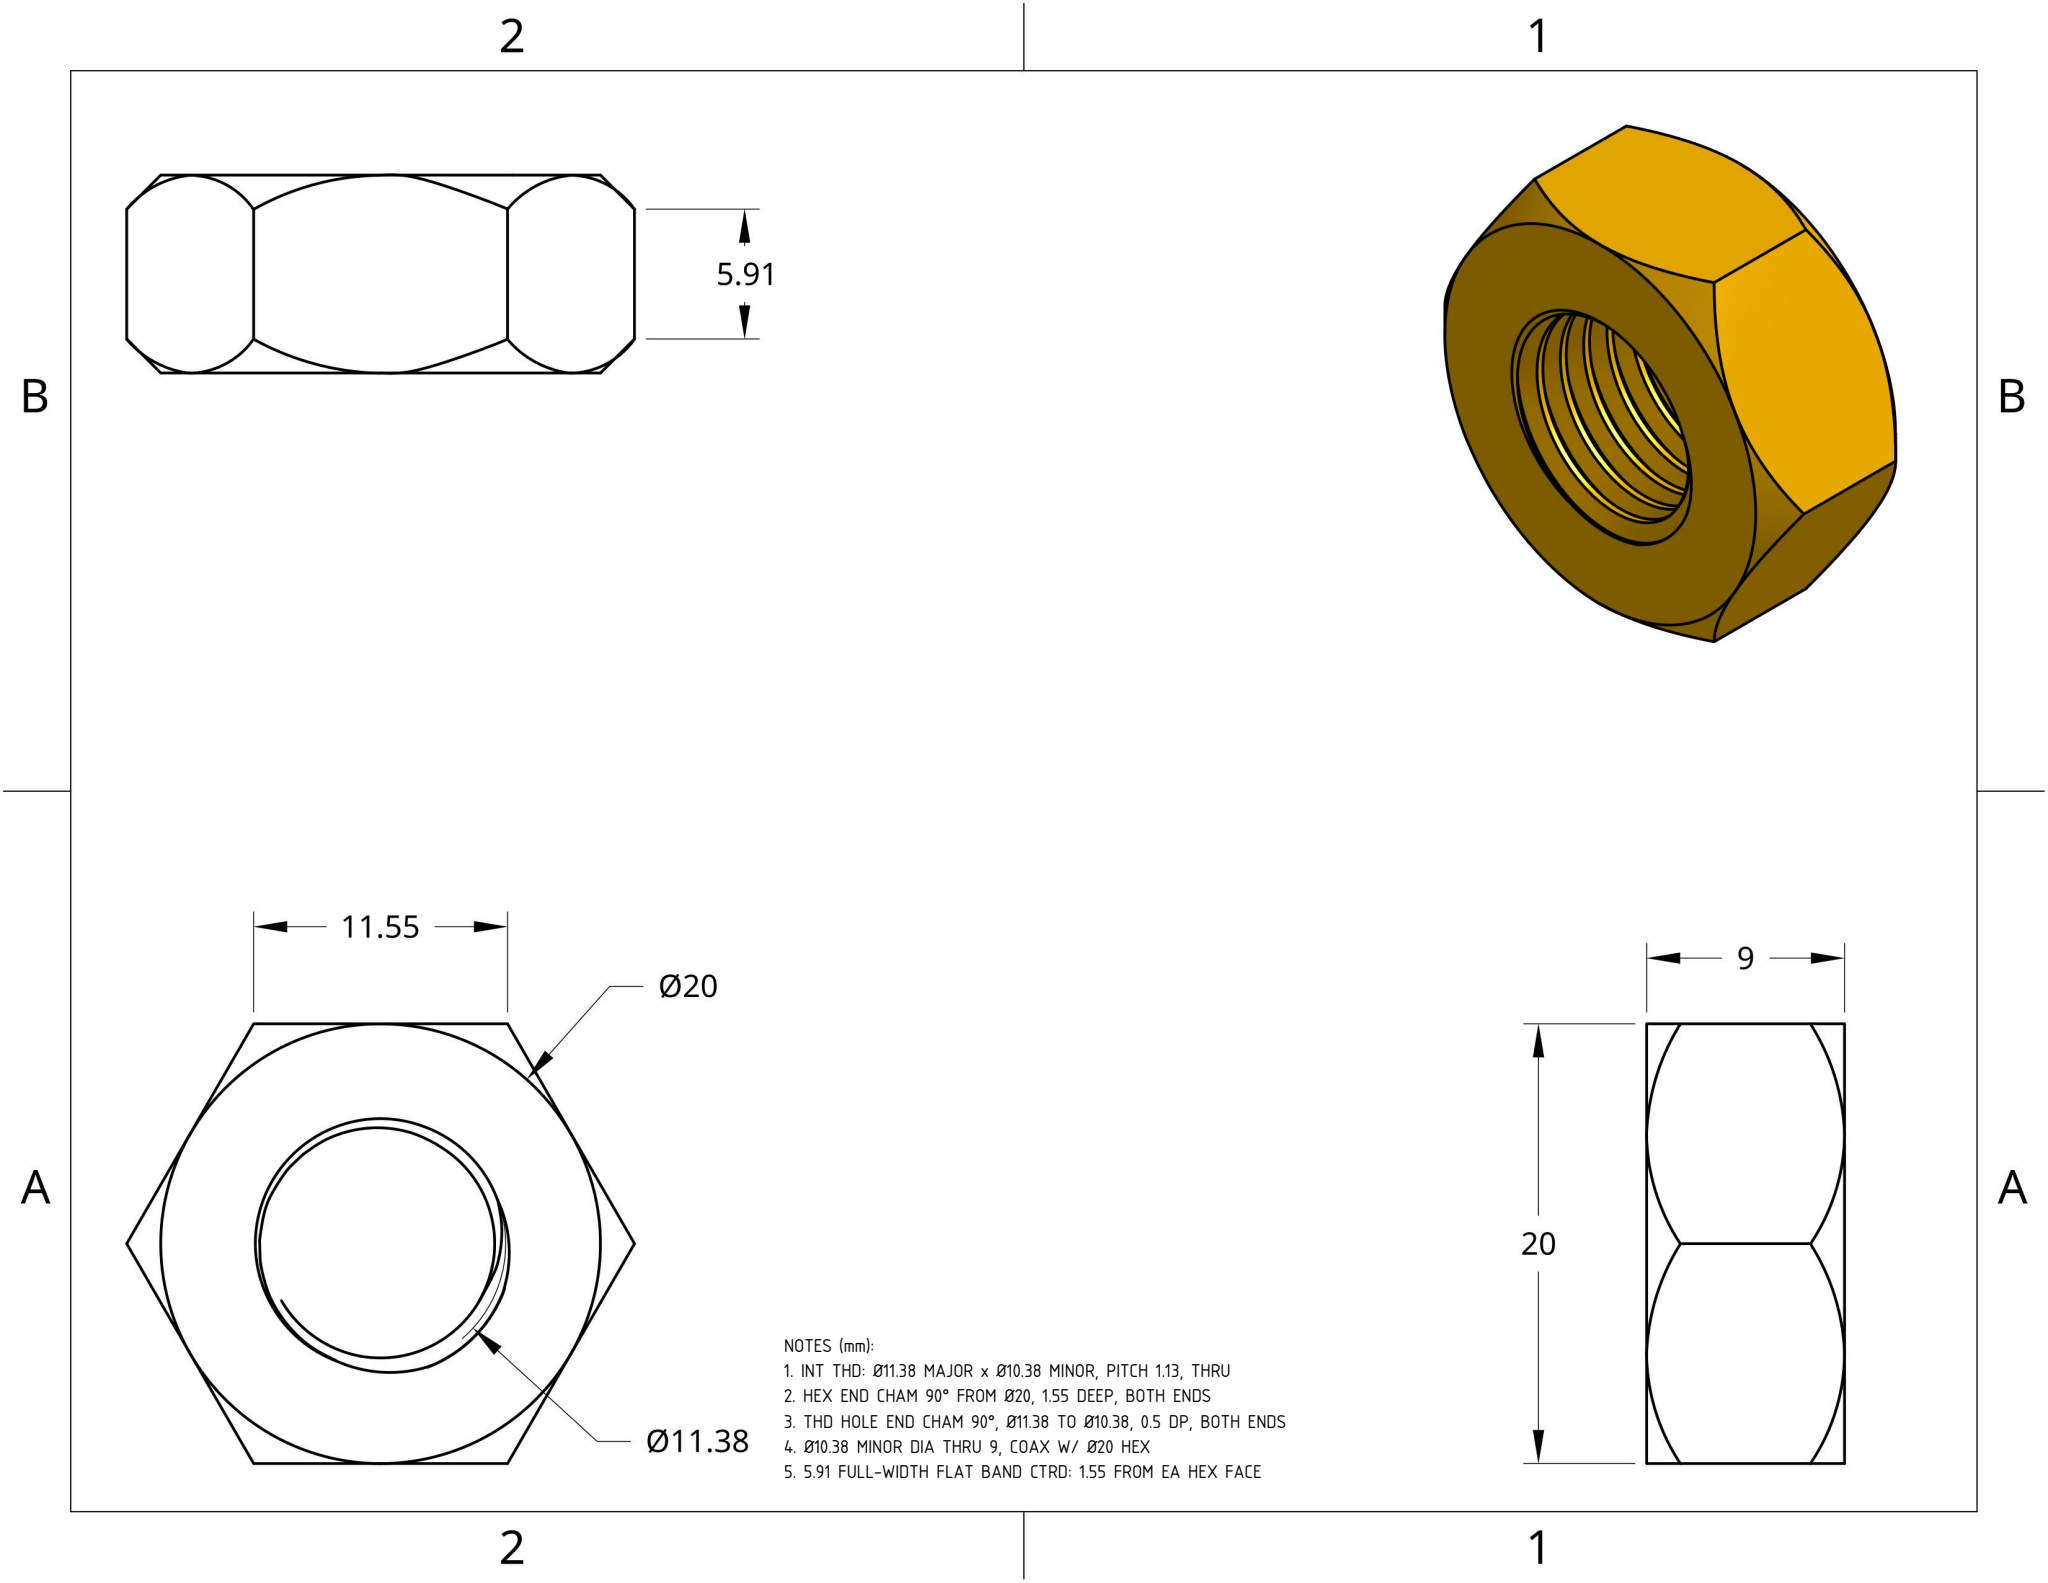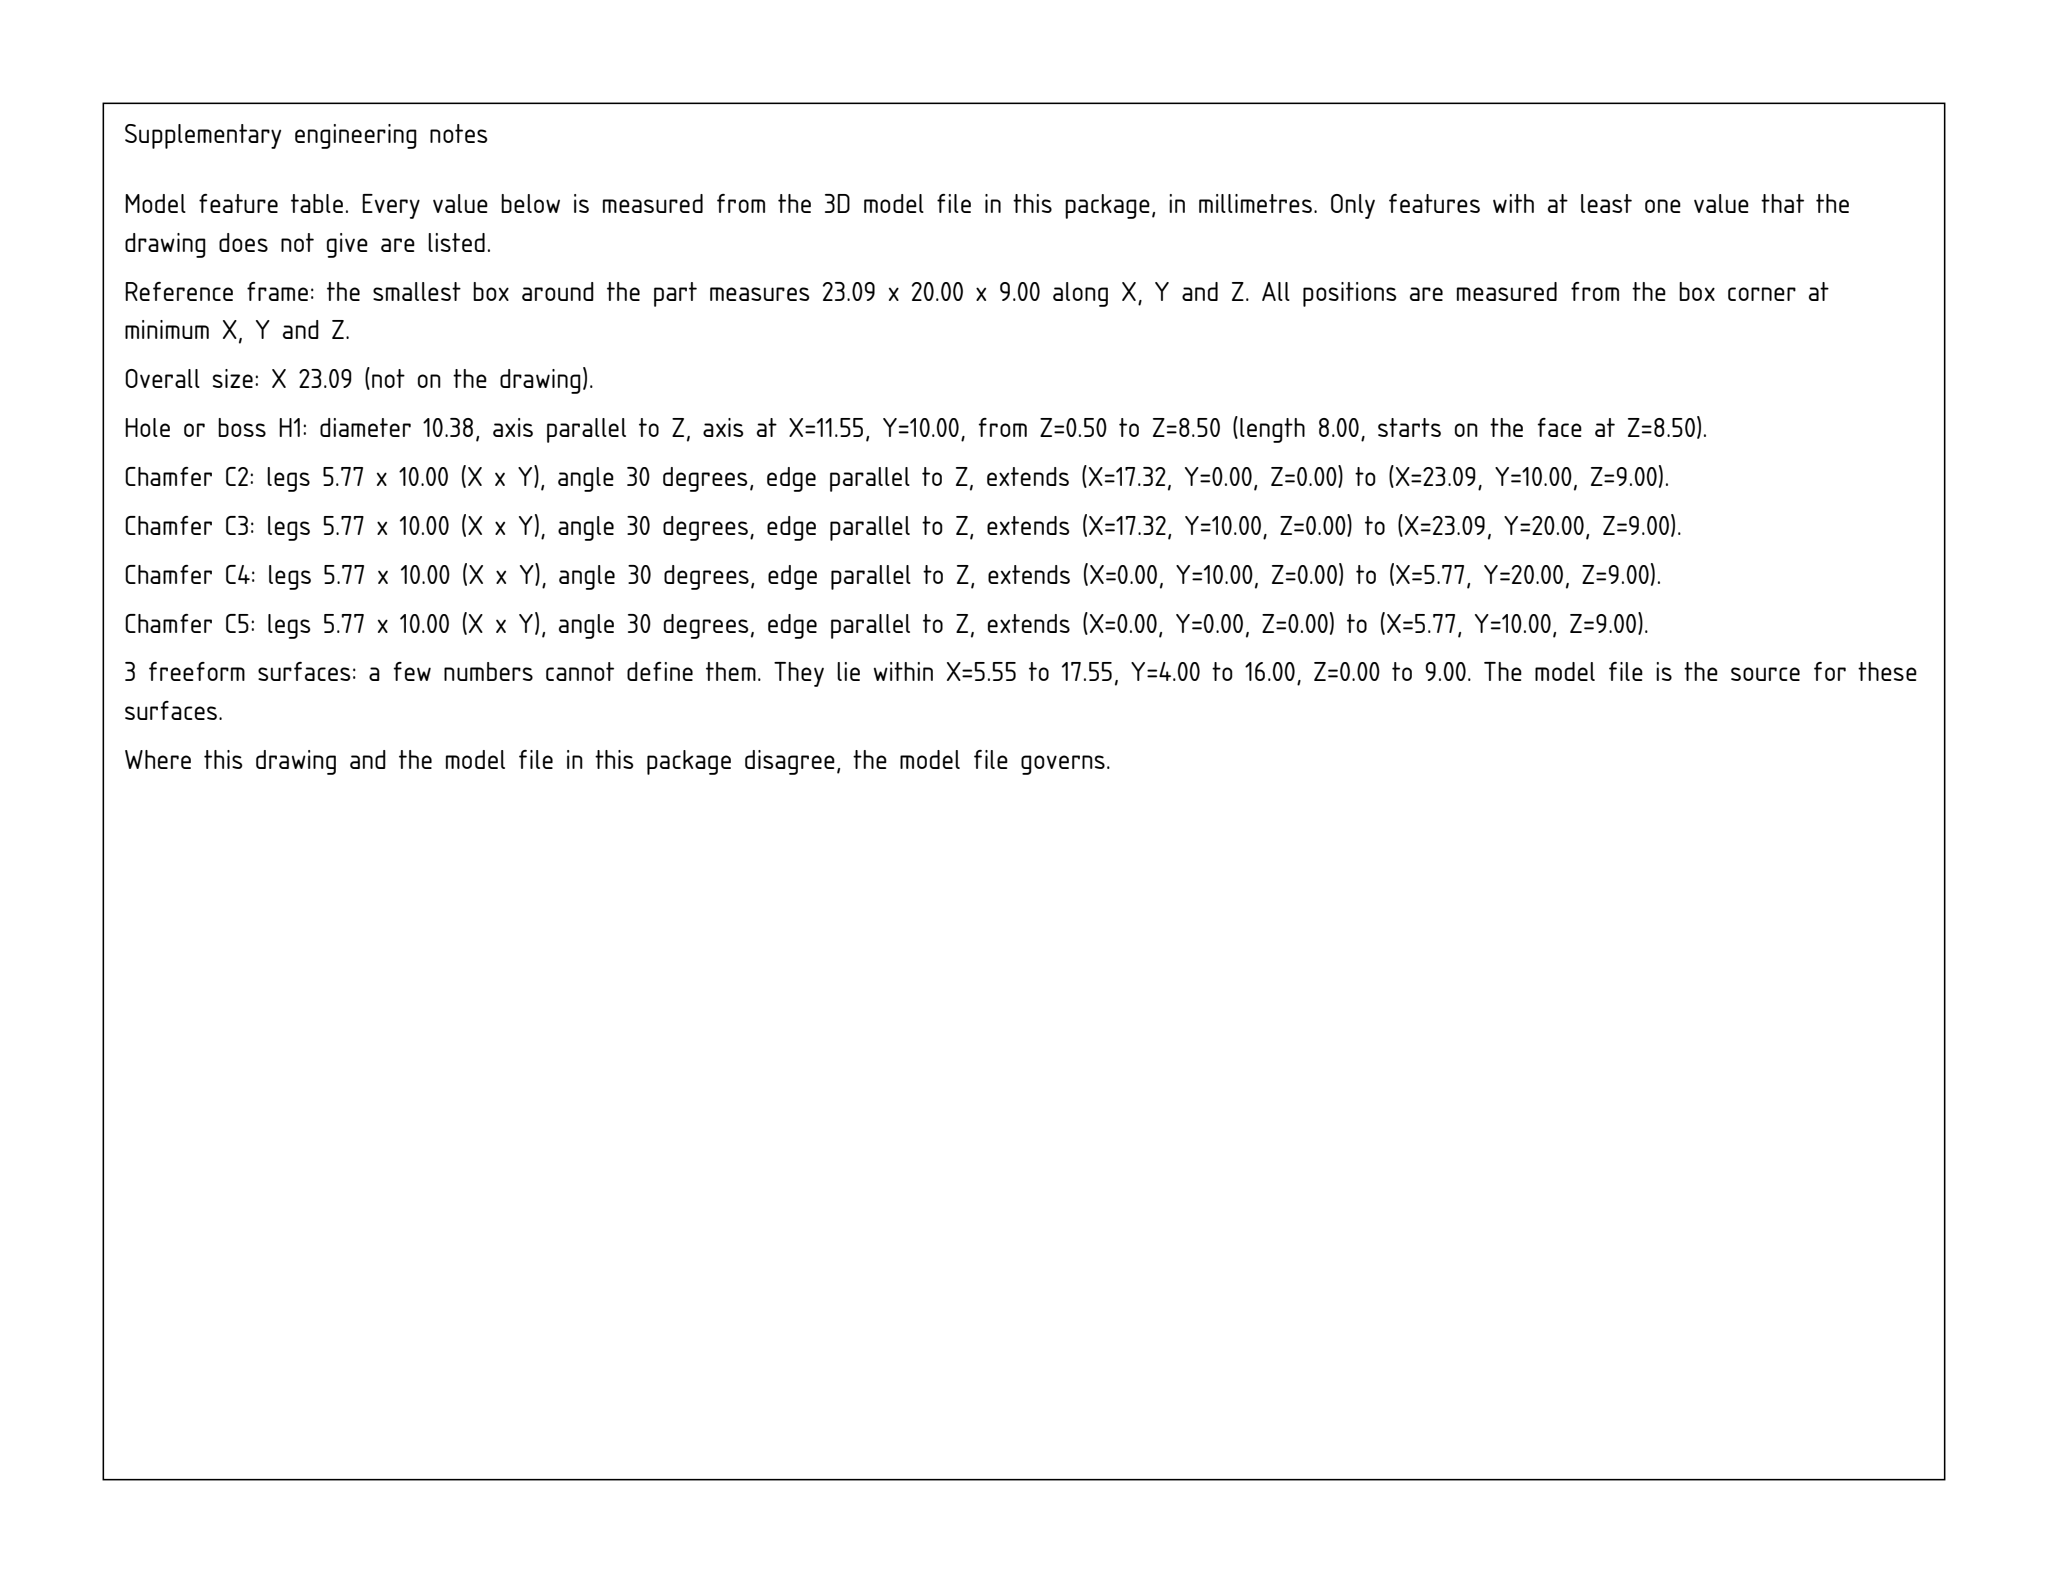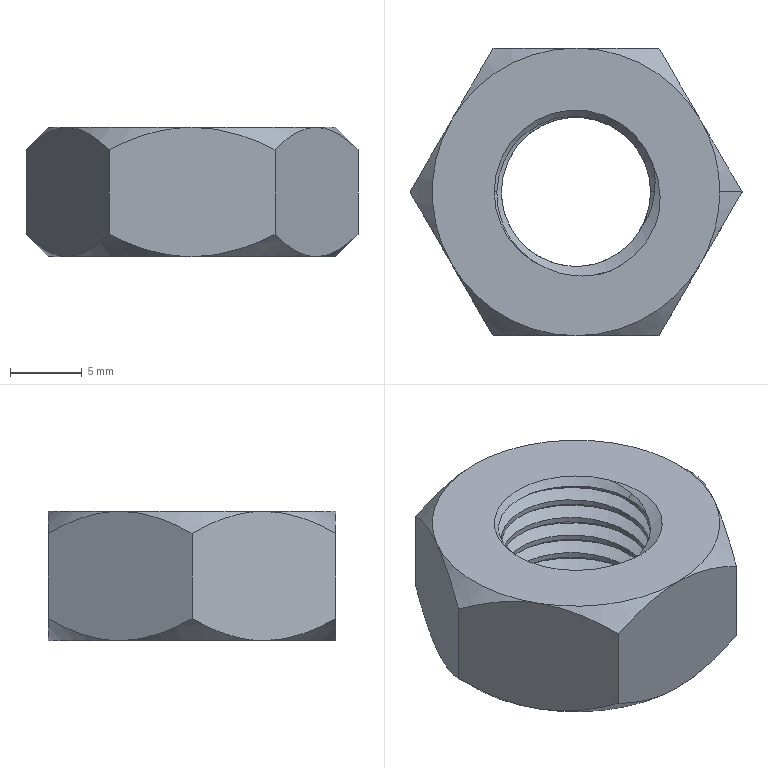Part | SolidWorks | mm | 1 solid | 42 faces | box 23.09 x 20 x 9 mm | volume 2213 mm3 | cone 19 | cylinder 12 | plane 8 | spline 3 | commonest cylinder face diameters 10.38 x12
Drawing notes:
INT THD: Ø11.38 MAJOR x Ø10.38 MINOR, PITCH 1.13, THRU | from the solid: Ø10.38 z-axis cylinders (9 segs x 1.13 lg + 1.0/0.63/0.25) at (11.55,11.55); cones ref dia 11.38 & 10.38; thd thru 9 thk (z 0.56 to 9.56)
HEX END CHAM 90° FROM Ø20, 1.55 DEEP, BOTH ENDS | from the solid: 14 cones incl angle 90° ref dia 20; (23.095-20)/2 = 1.55 depth per end; 9 - 2x1.55 = 5.91
THD HOLE END CHAM 90°, Ø11.38 TO Ø10.38, 0.5 DP, BOTH ENDS | from the solid: cones 90° ref dia 11.38 (2) and 10.38 (3); (11.38-10.38)/2 = 0.5
Ø10.38 MINOR DIA THRU 9, COAX W/ Ø20 HEX | from the solid: cylinders dia 10.38 axis z at pos (11.55,11.55), spanning hex thk 9 (z-planes 0.56 / 9.56)
5.91 FULL-WIDTH FLAT BAND CTRD: 1.55 FROM EA HEX FACE | from the solid: z-planes at 0.56 and 9.56 (9 thk); chamfer 1.55 each face leaves 5.905 band centered